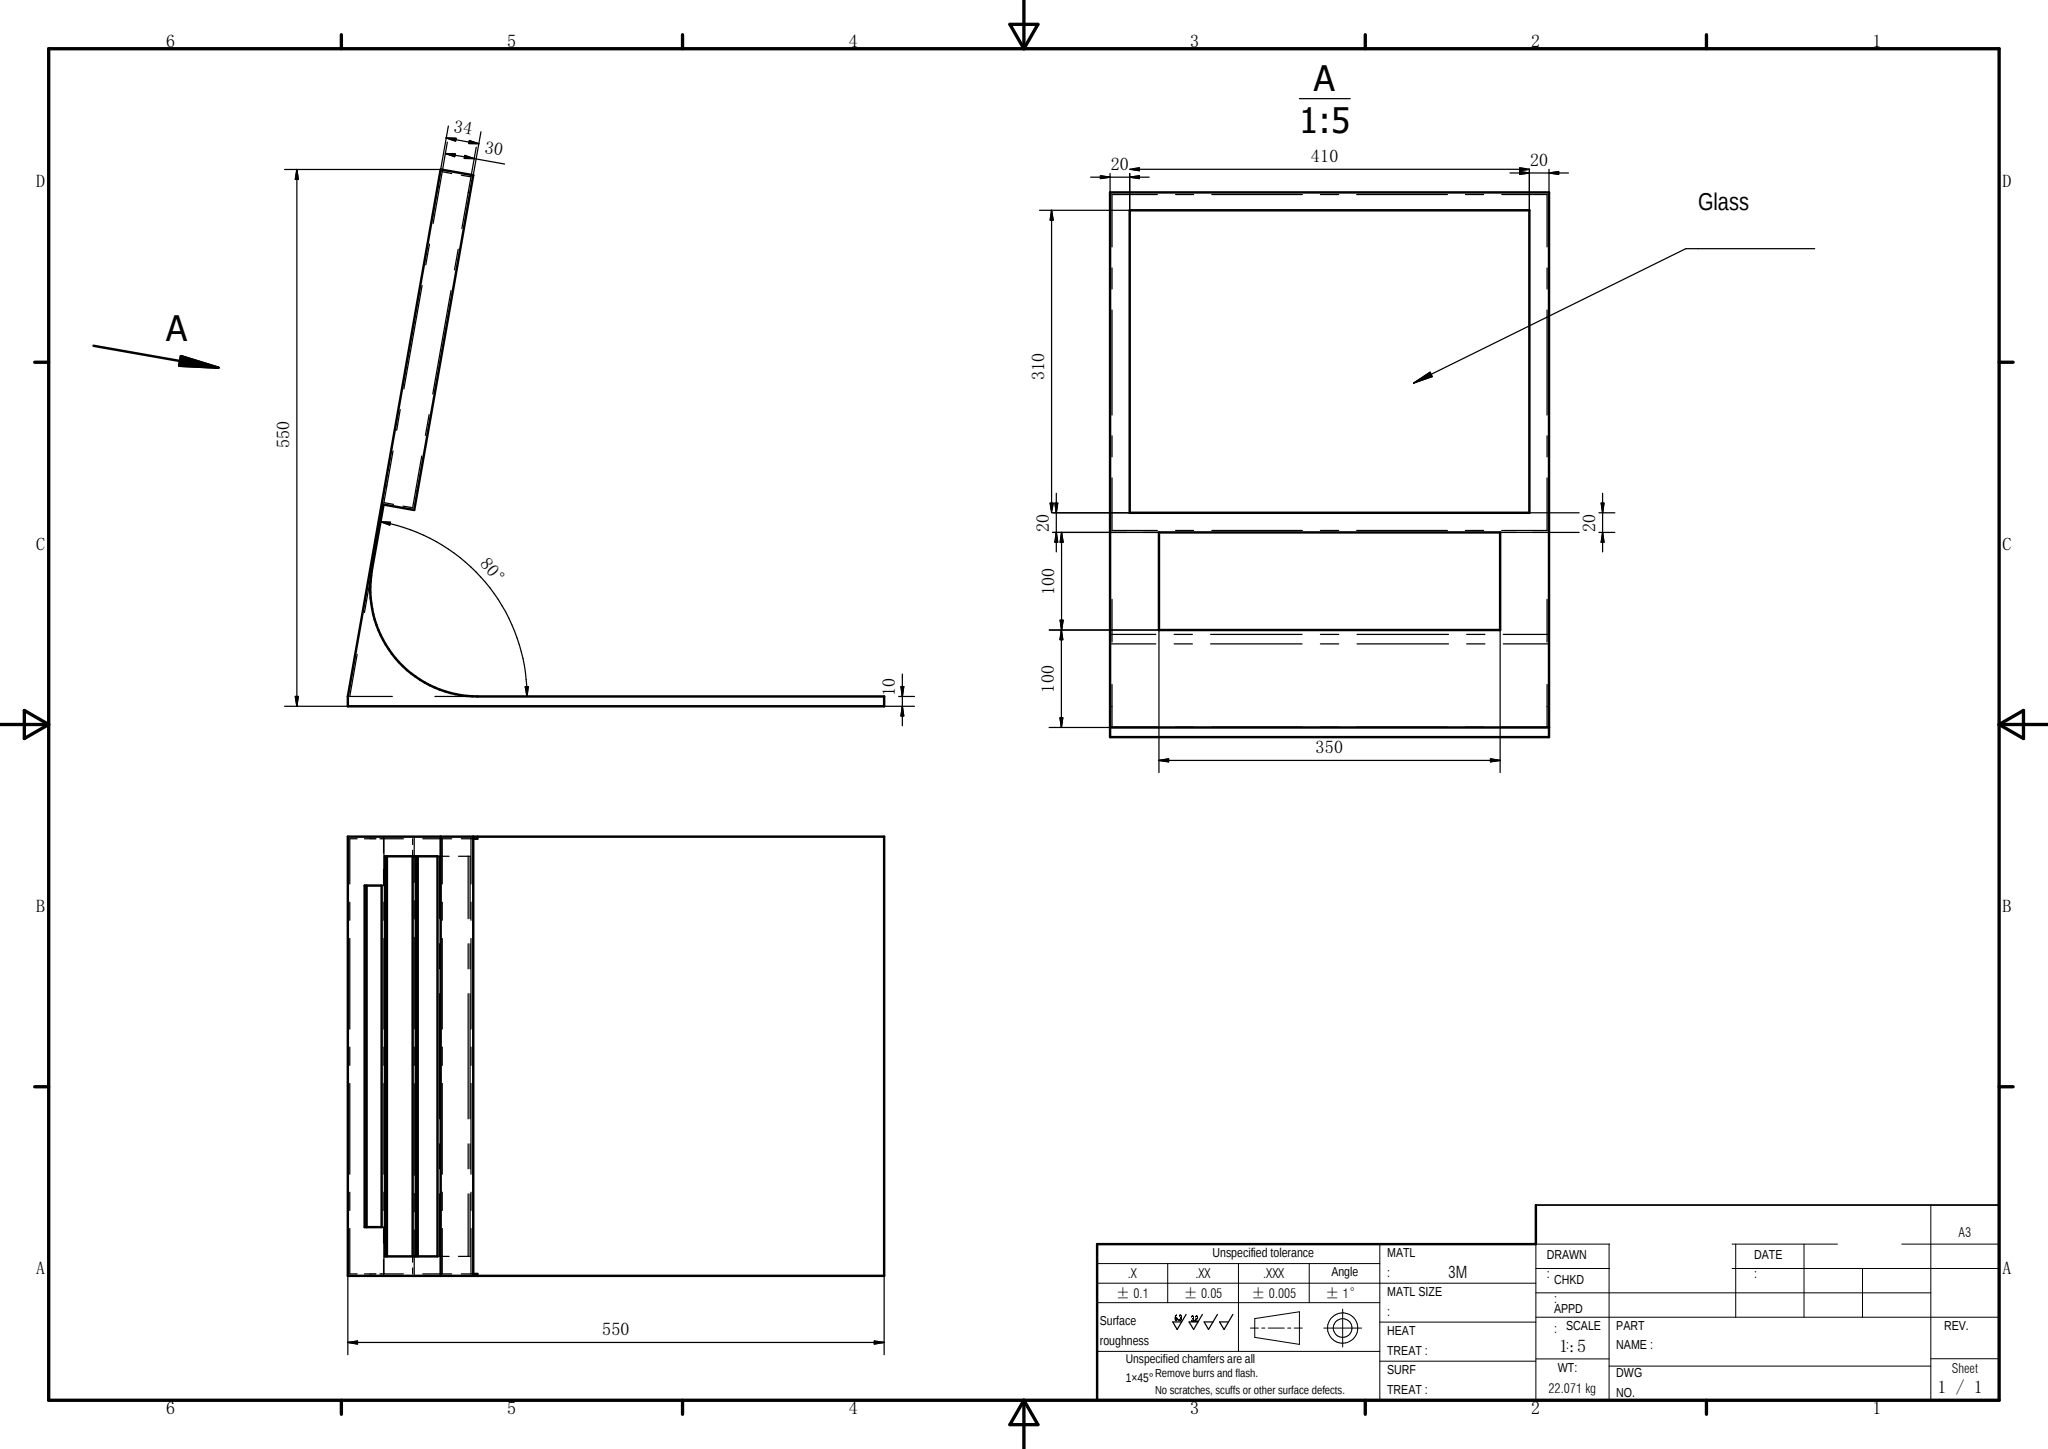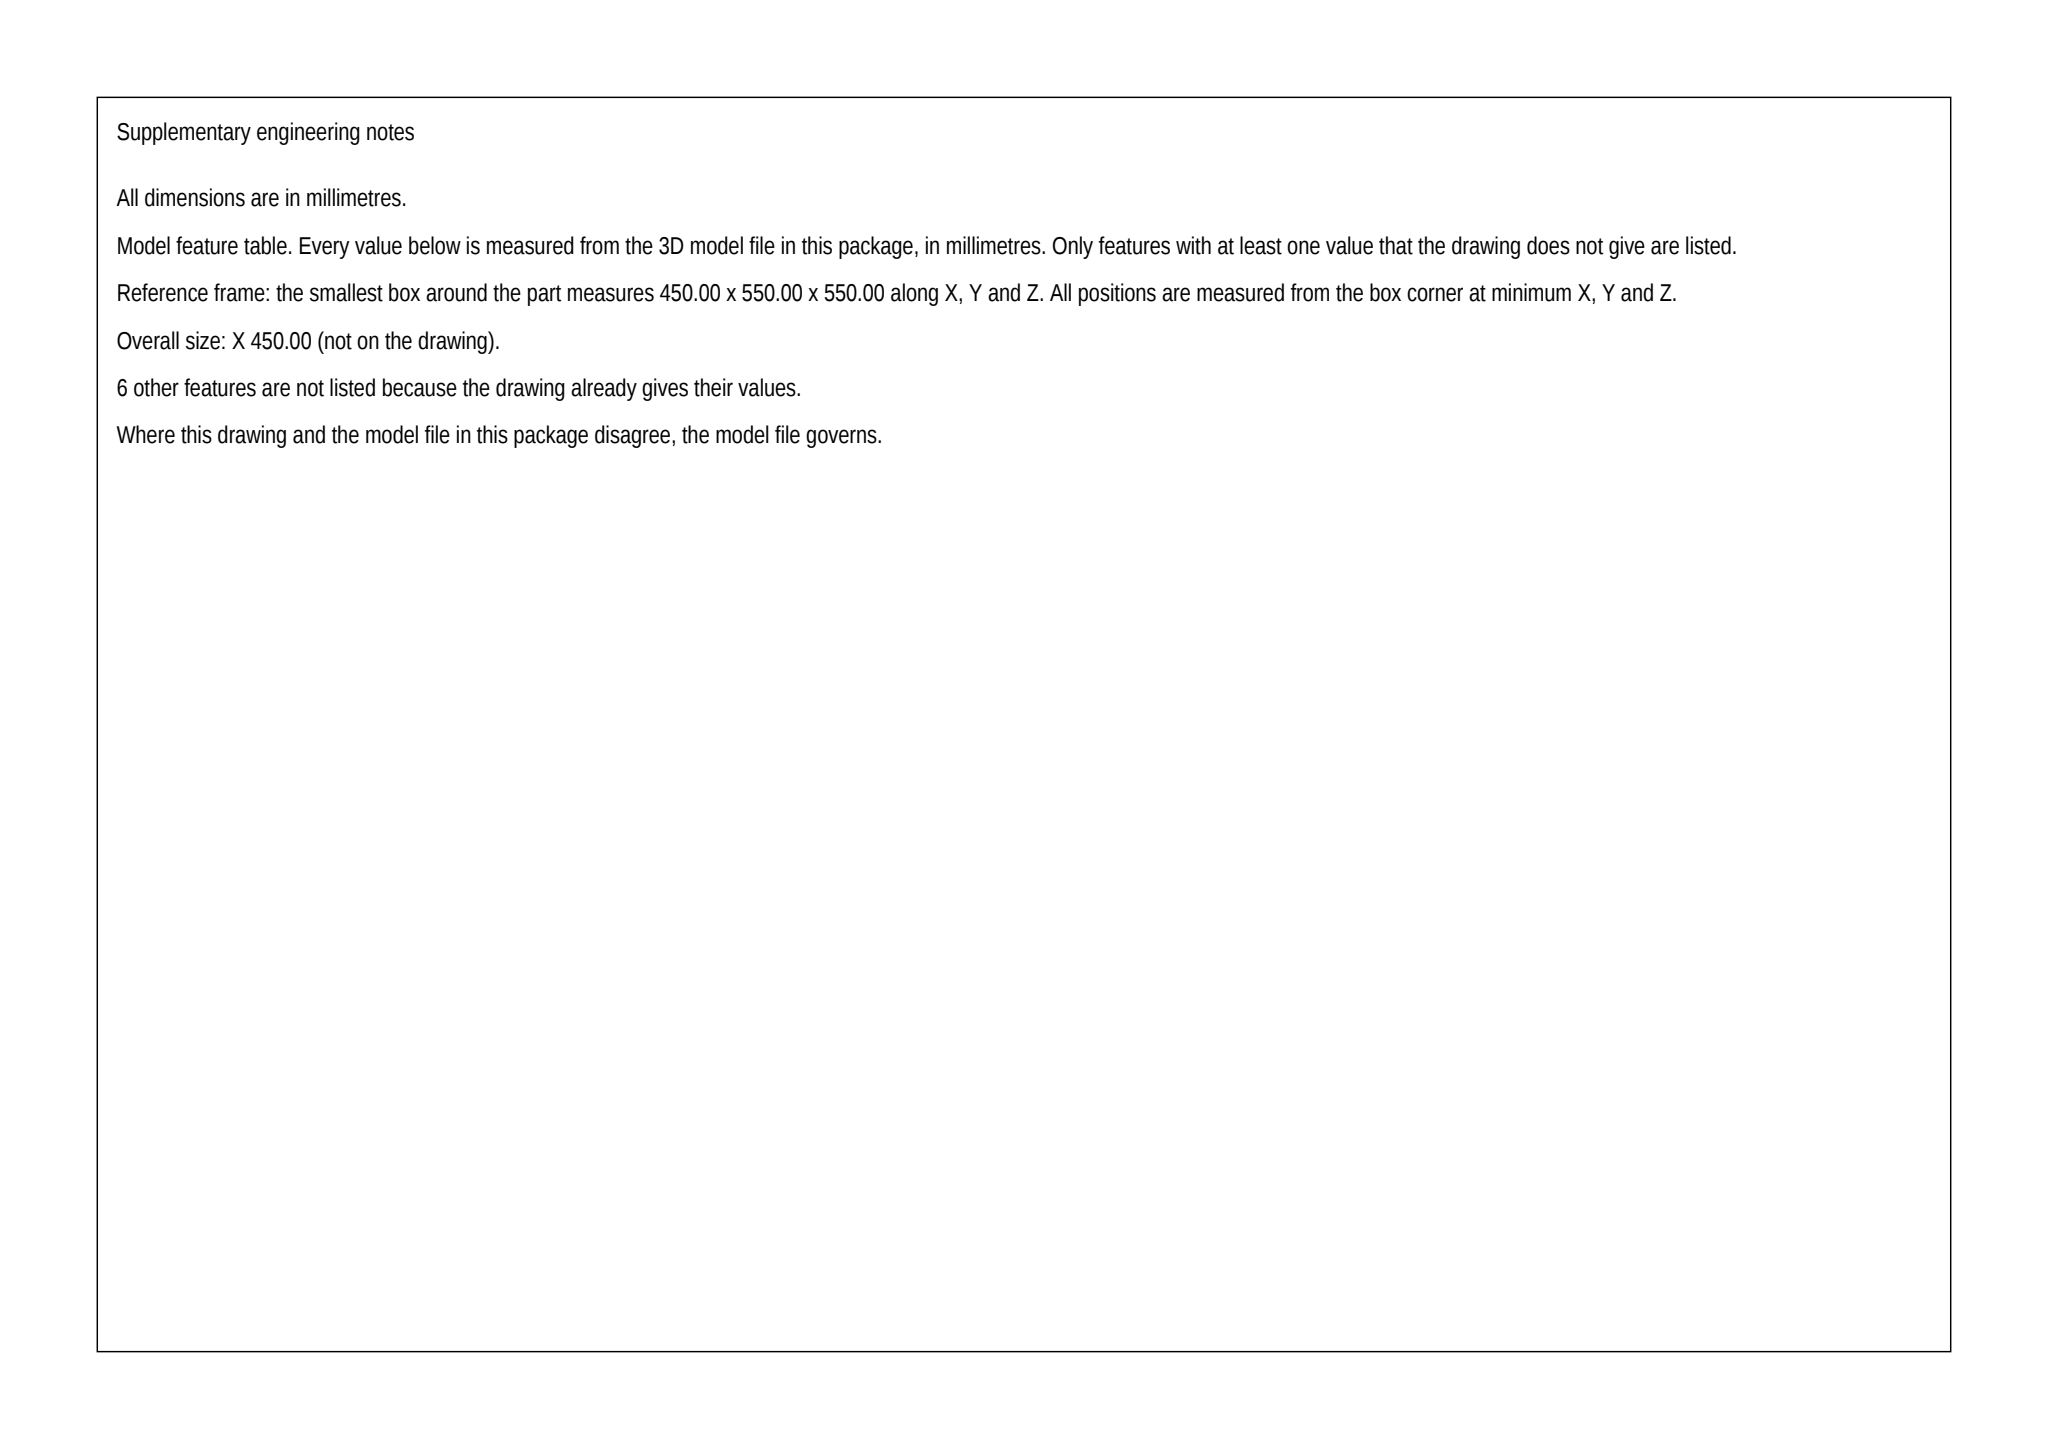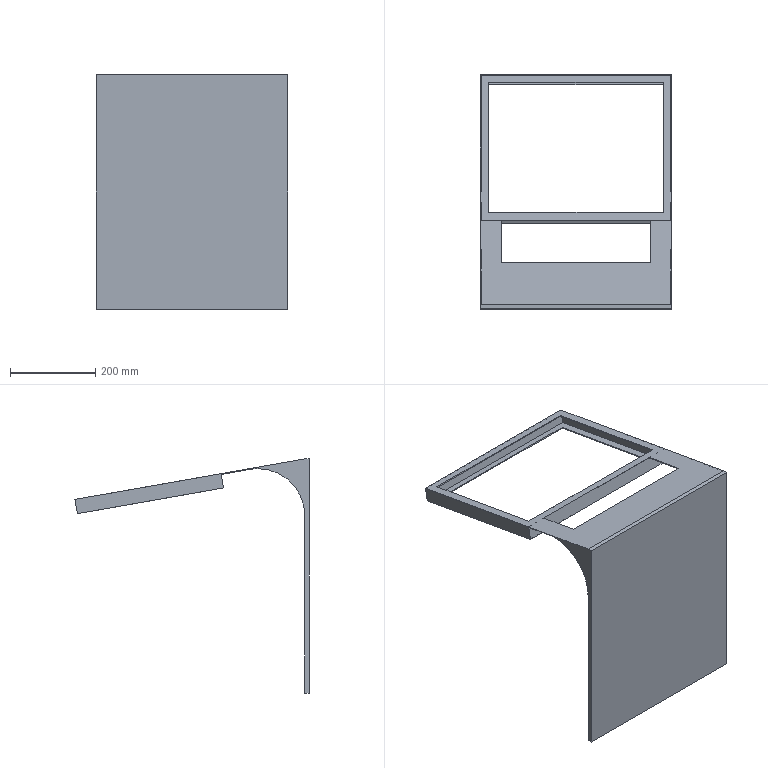Part | SolidWorks | mm | 1 solid | 34 faces | box 450 x 550 x 550 mm | volume 2811632 mm3 | plane 30 | cylinder 4 | commonest cylinder face diameters 220 x4
Drawing notes:
R110 TANGENT TO BASE 133.09 FROM PANEL-SIDE EDGE OF 550 BASE | from the solid: Cyl R110 (dia 220) axis at z=416.91, y=120, tangent to base top y=10; base z=0..550 => 550-416.91=133.09
GLASS RECESS: 2 DEEP STEP IN FRAME FRONT FACE, BOTH SIDES | from the solid: x planes at 0/2 and 448/450 give 2 mm step on each outer face of 450 wide frame
350 WIDE LOWER SECTION SYMM ABOUT CL, 50 FROM EA SIDE EDGE | from the solid: x planes 50 and 400 on 450 wide part: 400-50=350, 50 each side